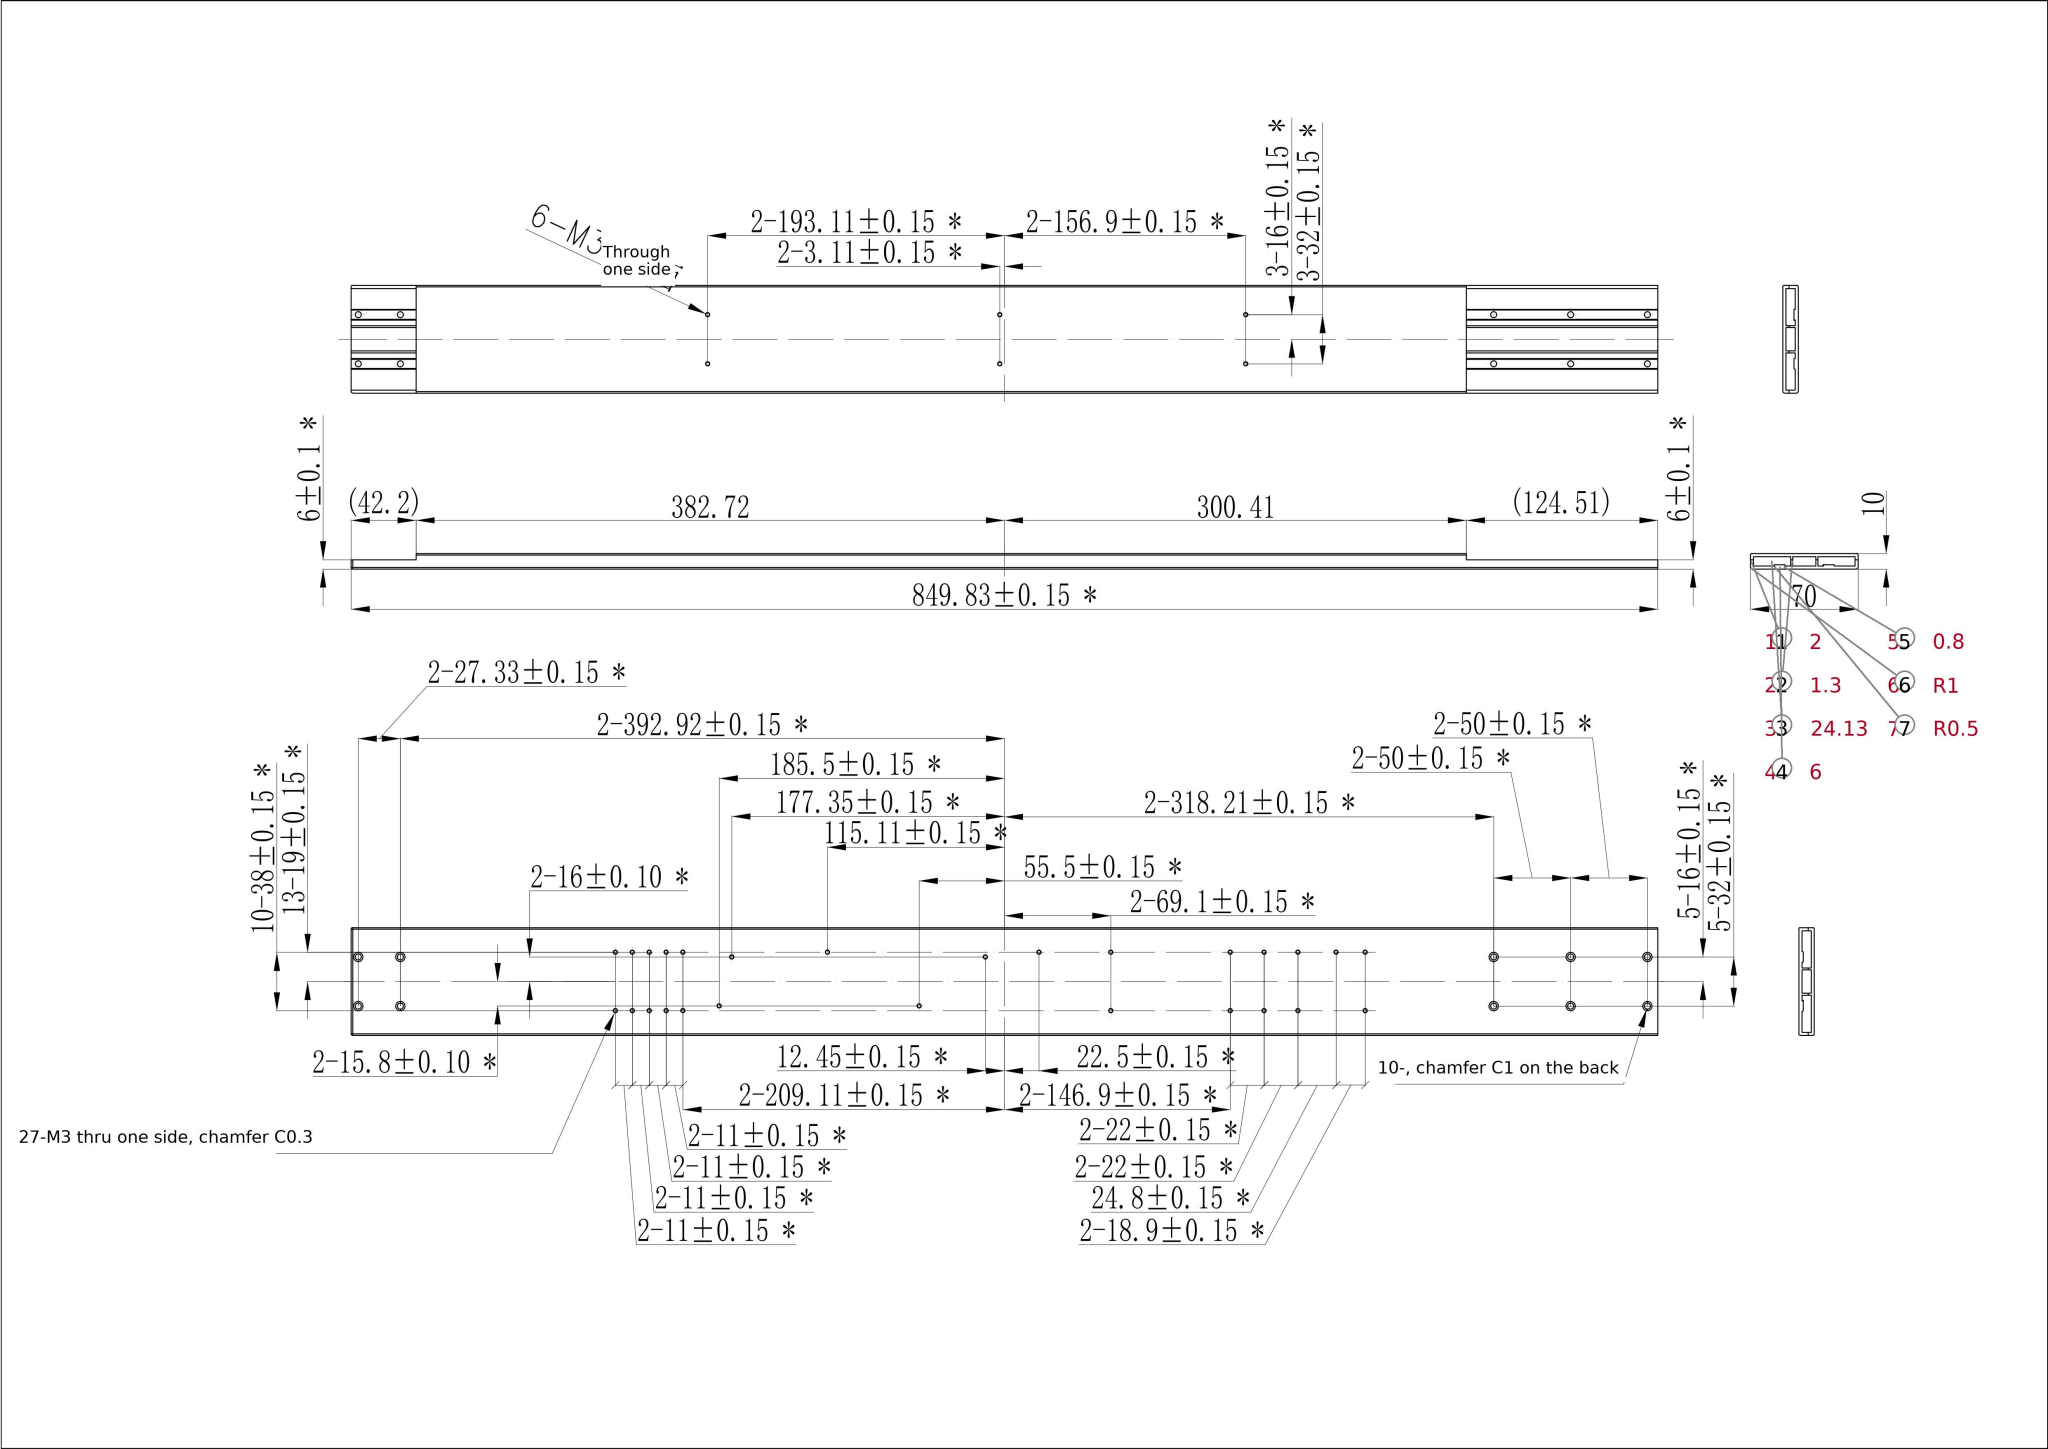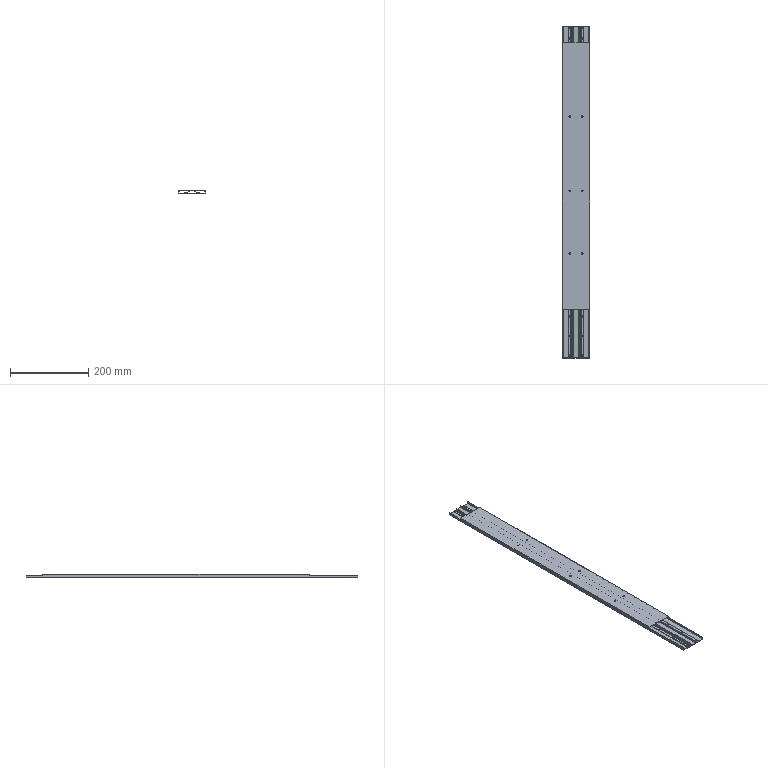Part | SolidWorks | mm | 1 solid | 281 faces | box 70 x 849.83 x 10 mm | volume 253690 mm3 | cylinder 126 | cone 86 | plane 65 | spline 4 | commonest cylinder face diameters 3 x66 1 x29 4 x20 2 x7 6.877 x4